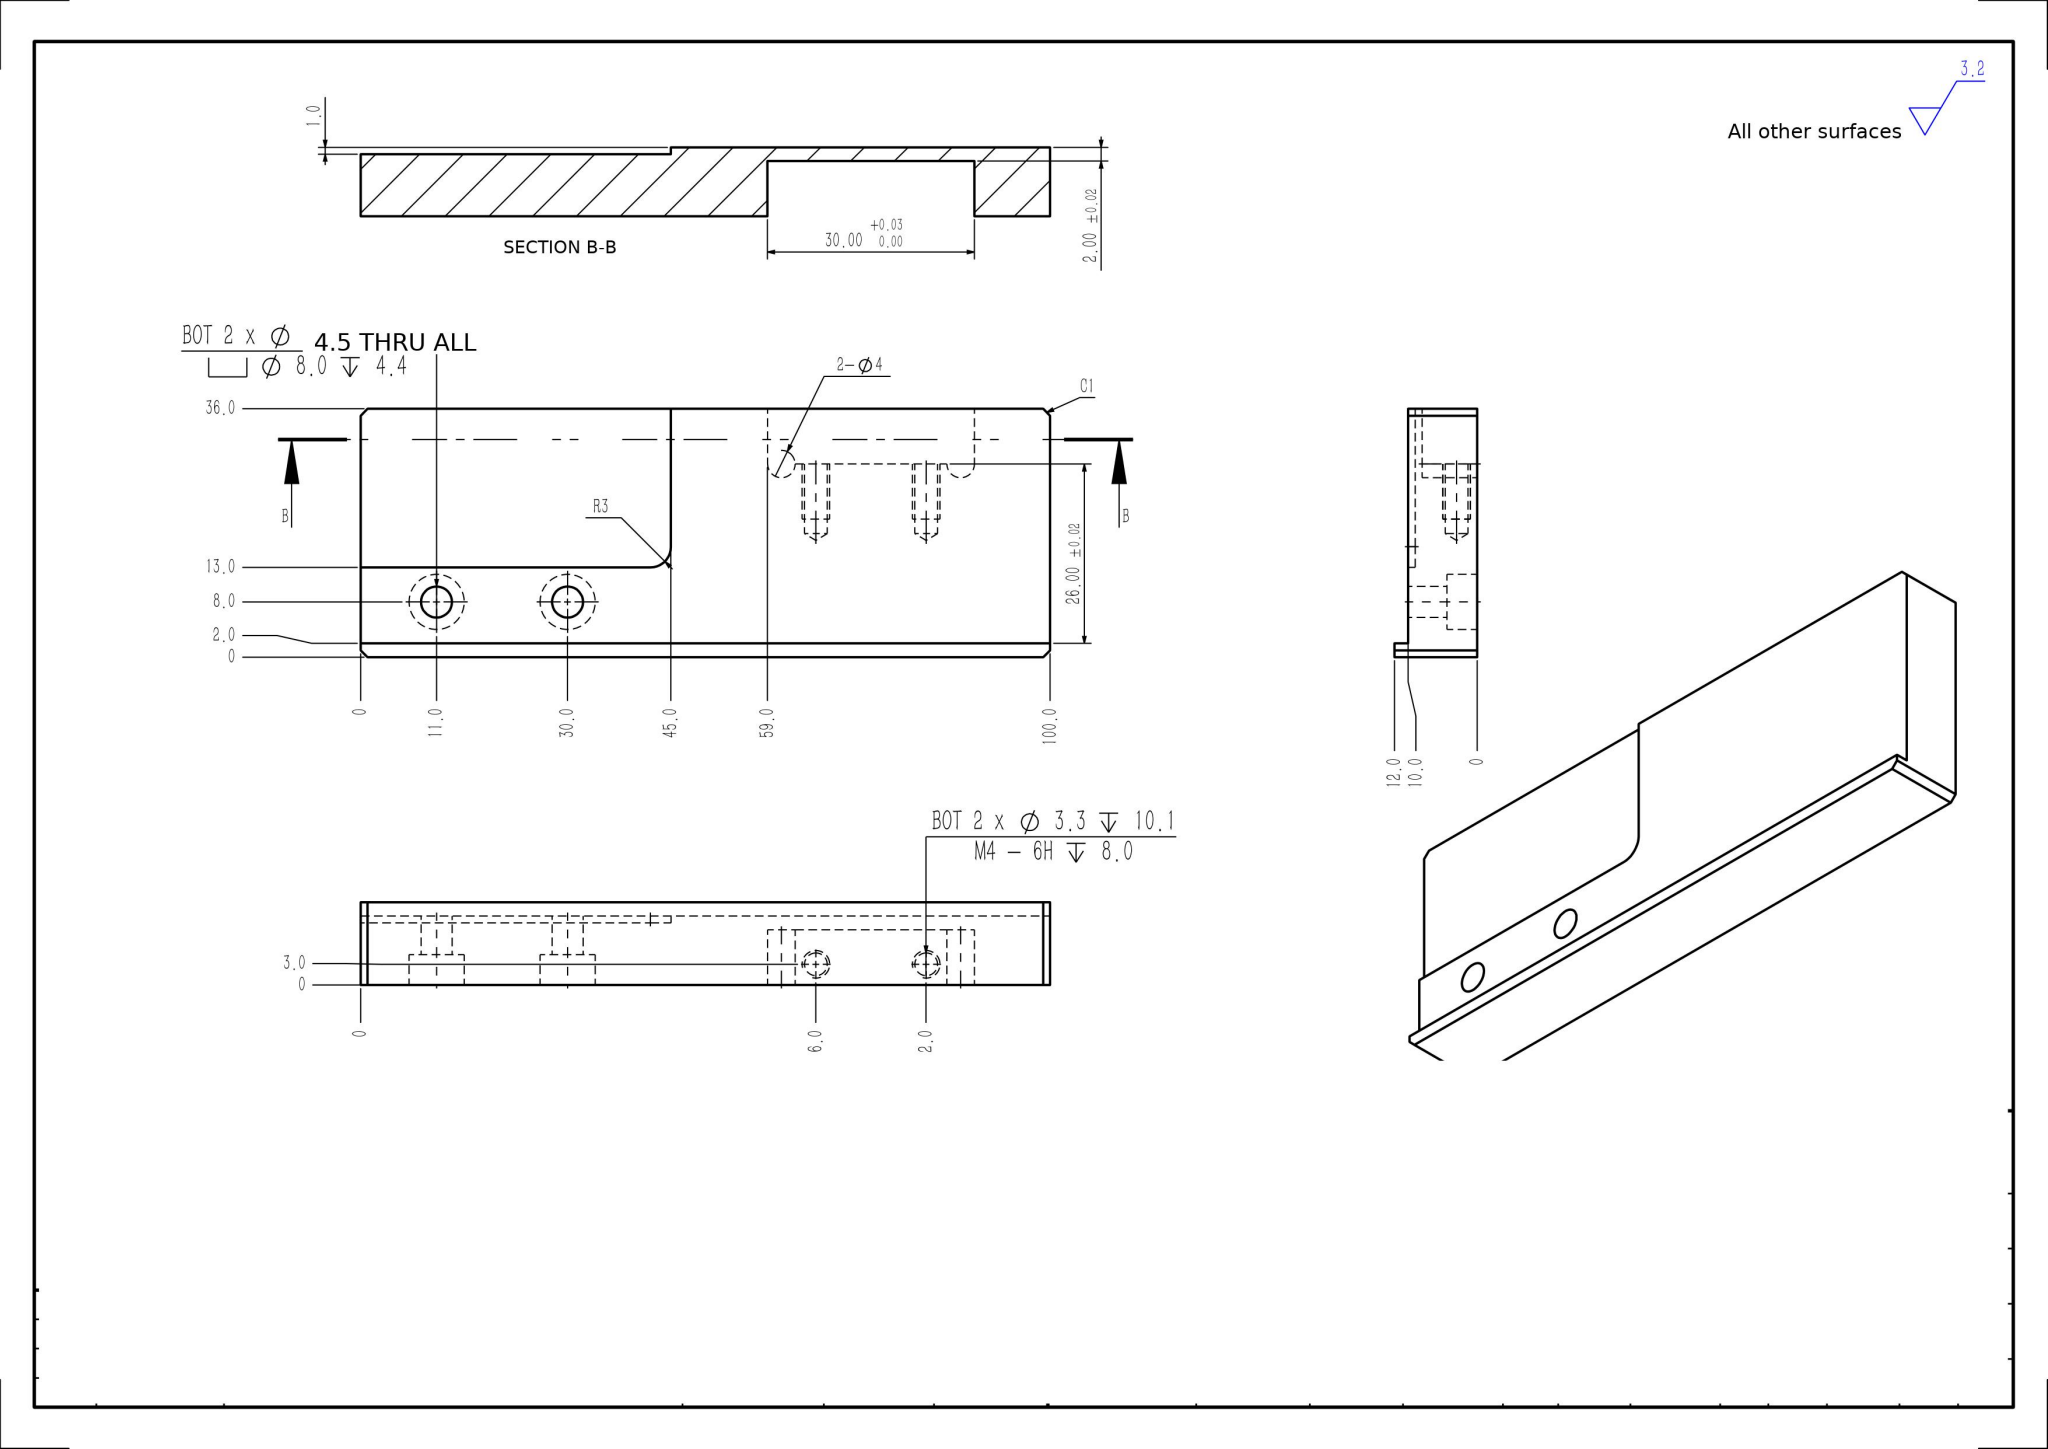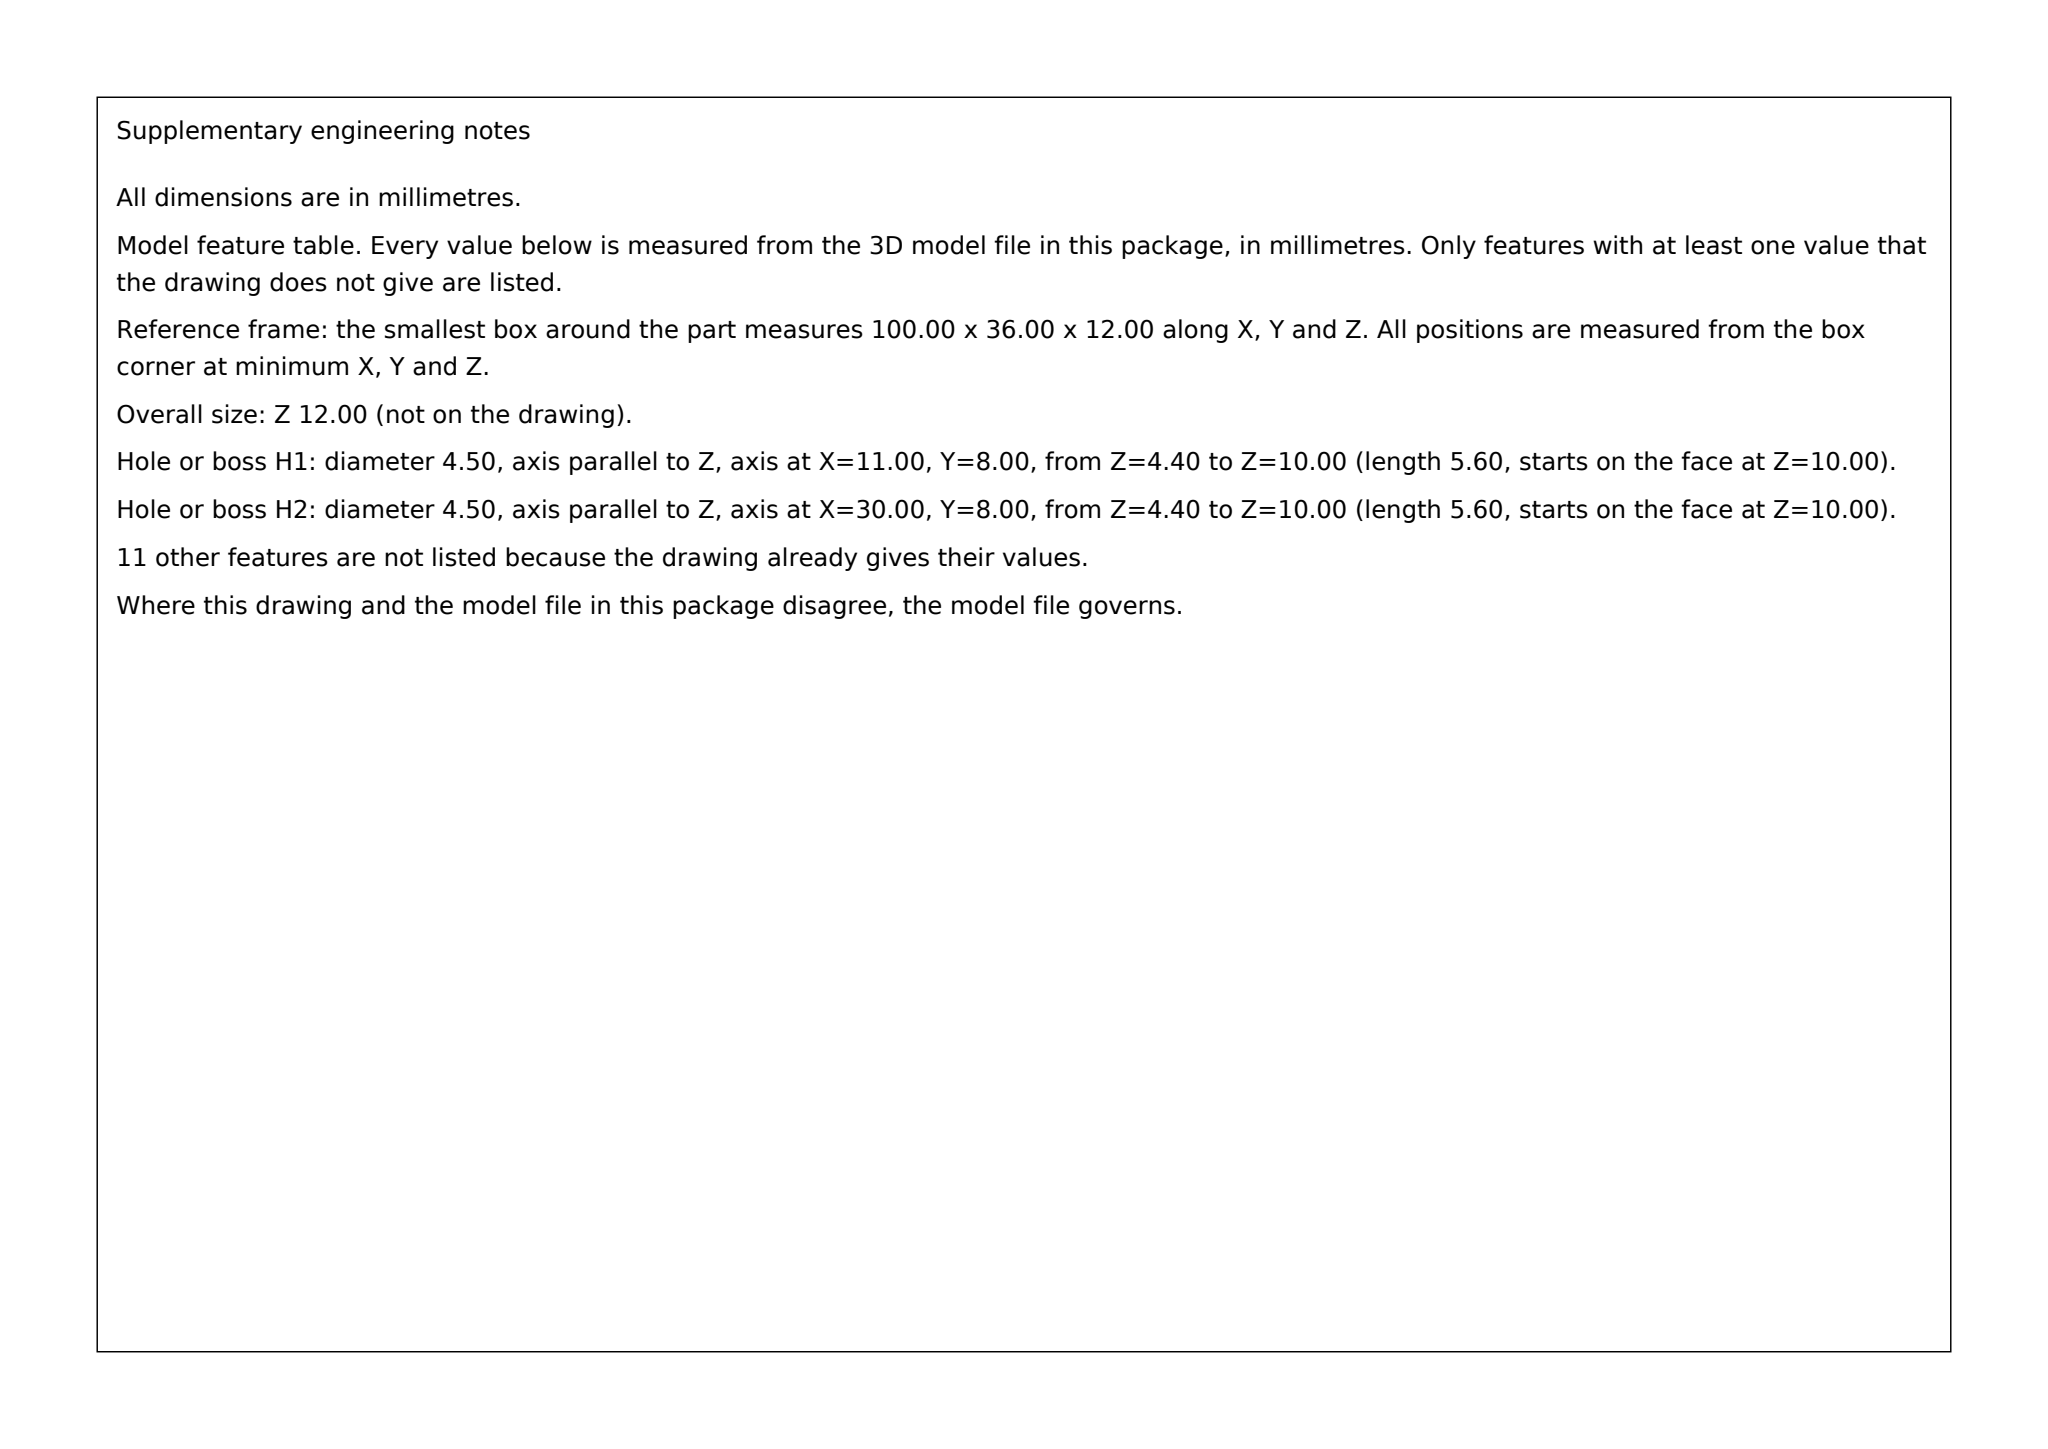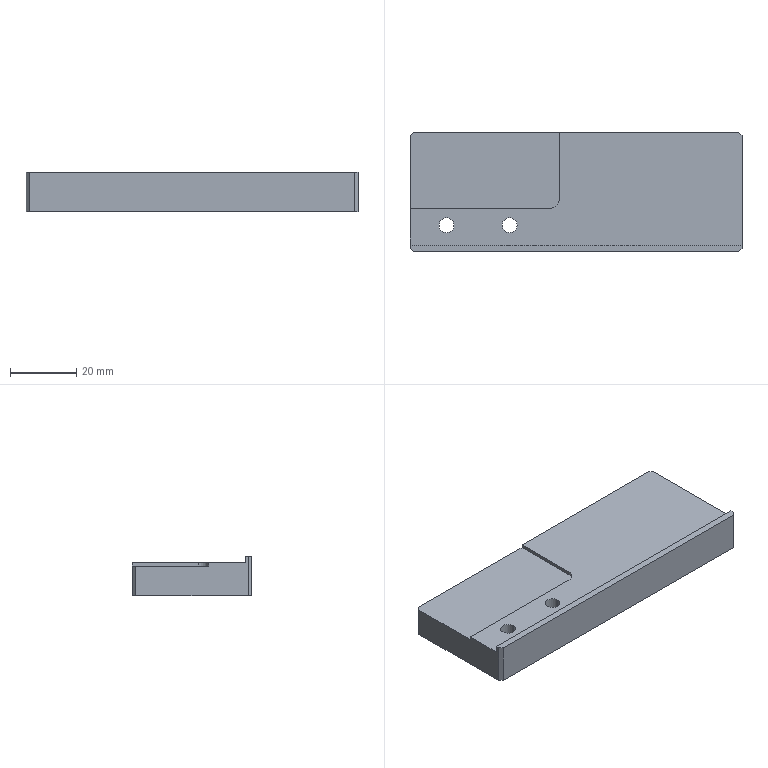Part | SolidWorks | mm | 1 solid | 40 faces | box 100 x 36 x 12 mm | volume 32526 mm3 | plane 21 | cylinder 15 | cone 4 | commonest cylinder face diameters 3.3 x4 8 x4 4.5 x4 4 x2 6 x1
build123d program:
from build123d import *

# Parameters (mm, degrees)
SKETCH1_W                                       = 100
SKETCH1_H                                       = 36
BOSS_EXTRUDE1_DEPTH                             = 6
SKETCH2_W                                       = 100
SKETCH2_H                                       = 34
CUT_EXTRUDE1_DEPTH                              = 2
CUT_EXTRUDE2_DEPTH                              = 1
SKETCH4_W                                       = 30
SKETCH4_H                                       = 8
CUT_EXTRUDE3_DEPTH                              = 8
SKETCH5_R                                       = 2
CUT_EXTRUDE4_DEPTH                              = 8
CHAMFER1_SIZE                                   = 1
M4_HEX_SOCKET_HEAD_CAP_SCREW_CBORE1_D           = 4.5
M4_HEX_SOCKET_HEAD_CAP_SCREW_CBORE1_CBORE_D     = 8
M4_HEX_SOCKET_HEAD_CAP_SCREW_CBORE1_CBORE_DEPTH = 4.4
M4_TAPPED_HOLE1_D                               = 3.3
M4_TAPPED_HOLE1_DEPTH                           = 10.1
M4_TAPPED_HOLE1_TIP                             = 0.9914


with BuildPart() as part:
    # Sketch1 → Boss-Extrude1 (new, symmetric)
    with BuildSketch(Plane.XY):
        Rectangle(SKETCH1_W, SKETCH1_H)
    extrude(amount=BOSS_EXTRUDE1_DEPTH, both=True)

    # Sketch2 → Cut-Extrude1 (cut)
    with BuildSketch(Plane.XY.offset(6)):
        with Locations((0, 1)):
            Rectangle(SKETCH2_W, SKETCH2_H)
    extrude(amount=-CUT_EXTRUDE1_DEPTH, mode=Mode.SUBTRACT)

    # Sketch3 → Cut-Extrude2 (cut)
    with BuildSketch(Plane.XY.offset(4)):
        with BuildLine():
            Line((-50, 18), (-5, 18))
            Line((-5, 18), (-5, -2))
            ThreePointArc((-5, -2), (-5.879, -4.121), (-8, -5))
            Line((-8, -5), (-50, -5))
            Line((-50, -5), (-50, 18))
        make_face()
    extrude(amount=-CUT_EXTRUDE2_DEPTH, mode=Mode.SUBTRACT)

    # Sketch4 → Cut-Extrude3 (cut)
    with BuildSketch(Plane(origin=(0, 18, 0), x_dir=(1, 0, 0), z_dir=(0, 1, 0))):
        with Locations((24, 2)):
            Rectangle(SKETCH4_W, SKETCH4_H)
    extrude(amount=-CUT_EXTRUDE3_DEPTH, mode=Mode.SUBTRACT)

    # Sketch5 → Cut-Extrude4 (cut)
    with BuildSketch(Plane(origin=(0, 0, -6), x_dir=(-1, 0, 0), z_dir=(0, 0, -1))):
        with Locations((-11, 10)):
            Circle(SKETCH5_R)
        with Locations((-37, 10)):
            Circle(SKETCH5_R)
    extrude(amount=-CUT_EXTRUDE4_DEPTH, mode=Mode.SUBTRACT)

    # Chamfer1
    chamfer1_edges = [part.edges().sort_by_distance(p)[0] for p in [
        (50, -18, 0),
        (-50, -18, 0),
        (50, 18, -1),
        (-50, 18, -1.5),
    ]]
    chamfer(chamfer1_edges, length=CHAMFER1_SIZE)

    # M4 Hex Socket Head Cap Screw CBORE1 (through all)
    with Locations(Plane(origin=(0, 0, -6), x_dir=(-1, 0, 0), z_dir=(0, 0, -1))):
        with Locations((39, -10), (20, -10)):
            CounterBoreHole(M4_HEX_SOCKET_HEAD_CAP_SCREW_CBORE1_D / 2, M4_HEX_SOCKET_HEAD_CAP_SCREW_CBORE1_CBORE_D / 2, M4_HEX_SOCKET_HEAD_CAP_SCREW_CBORE1_CBORE_DEPTH)

    # M4 Tapped Hole1
    with Locations(Plane(origin=(0, 10, 0), x_dir=(1, 0, 0), z_dir=(0, 1, 0))):
        with Locations((16, 3), (32, 3)):
            Hole(M4_TAPPED_HOLE1_D / 2, depth=M4_TAPPED_HOLE1_DEPTH)
            with Locations((0, 0, -(M4_TAPPED_HOLE1_DEPTH + M4_TAPPED_HOLE1_TIP / 2))):  # 118° drill point
                Cone(0, M4_TAPPED_HOLE1_D / 2, M4_TAPPED_HOLE1_TIP, mode=Mode.SUBTRACT)


solid = part.part